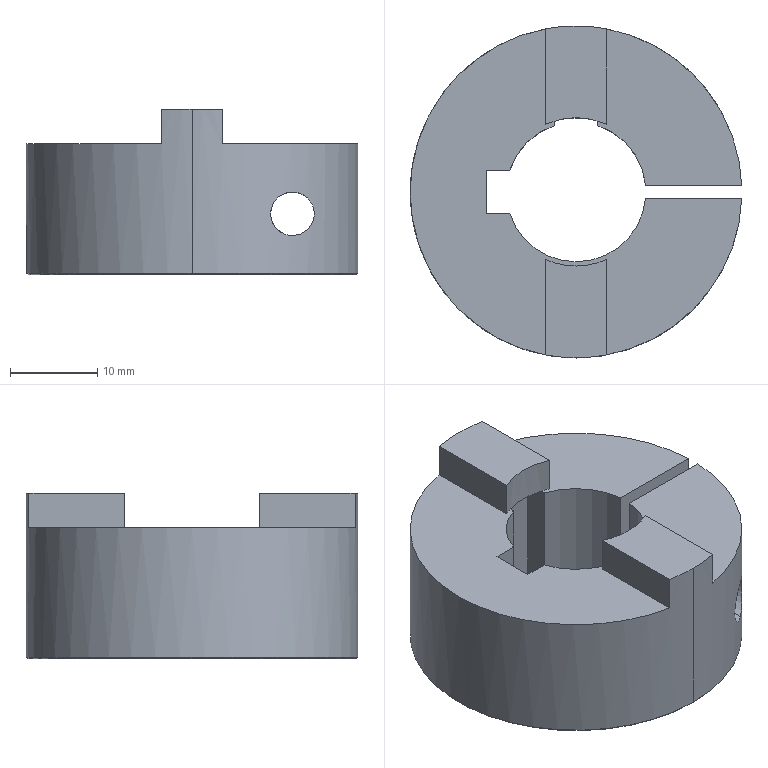Component | SolidWorks | ServoDriveMotorModule-1_MCOCGWK38_16_16-1_MCOCGXK3816-2 | 1 solid | 40 faces | volume 13168 mm3 | plane 19 | cylinder 16 | cone 5 | commonest cylinder face diameters 5 x4 16 x4 17 x3 38 x3 8.6 x2 | material AISI 1045 Steel, cold drawn